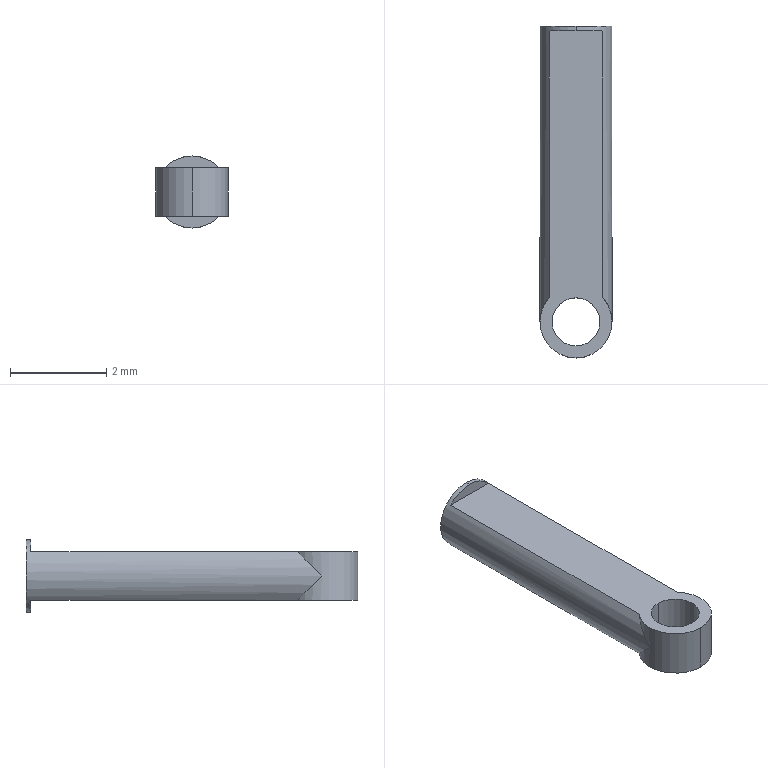Component | SolidWorks | ConnectingRodRockerArm-10 | 1 solid | 17 faces | box 1.5 x 6.9 x 1.5 mm | volume 6 mm3 | cylinder 10 | plane 7 | commonest cylinder face diameters 1.5 x4 1 x2 0.7 x2 0.8 x2
STEP:
#1=COLOUR_RGB('',0.7922,0.8196,0.9333);
#2=FILL_AREA_STYLE_COLOUR('',#1);
#3=FILL_AREA_STYLE('',(#2));
#4=SURFACE_STYLE_FILL_AREA(#3);
#5=SURFACE_SIDE_STYLE('',(#4));
#6=SURFACE_STYLE_USAGE(.BOTH.,#5);
#7=PRESENTATION_STYLE_ASSIGNMENT((#6));
#8=CARTESIAN_POINT('',(0.3877,0.1328,0.2657));
#9=VERTEX_POINT('',#8);
#10=CARTESIAN_POINT('',(0.3877,0.1328,0.3248));
#11=VERTEX_POINT('',#10);
#12=CARTESIAN_POINT('',(0.3877,0.1328,0.2953));
#13=DIRECTION('',(-0.,1.,-0.));
#14=DIRECTION('',(0.,0.,-1.));
#15=AXIS2_PLACEMENT_3D('',#12,#13,#14);
#16=CIRCLE('',#15,0.02953);
#17=EDGE_CURVE('',#9,#11,#16,.T.);
#18=ORIENTED_EDGE('',*,*,#17,.F.);
#19=CARTESIAN_POINT('',(0.3877,0.1289,0.2657));
#20=VERTEX_POINT('',#19);
#21=CARTESIAN_POINT('',(0.3877,0.1289,0.2657));
#22=DIRECTION('',(0.,-1.,0.));
#23=VECTOR('',#22,39.37);
#24=LINE('',#21,#23);
#25=EDGE_CURVE('',#9,#20,#24,.T.);
#26=ORIENTED_EDGE('',*,*,#25,.T.);
#27=CARTESIAN_POINT('',(0.3657,0.1289,0.2756));
#28=VERTEX_POINT('',#27);
#29=CARTESIAN_POINT('',(0.3877,0.1289,0.2953));
#30=DIRECTION('',(-0.,1.,-0.));
#31=DIRECTION('',(0.,0.,-1.));
#32=AXIS2_PLACEMENT_3D('',#29,#30,#31);
#33=CIRCLE('',#32,0.02953);
#34=EDGE_CURVE('',#20,#28,#33,.T.);
#35=ORIENTED_EDGE('',*,*,#34,.T.);
#36=CARTESIAN_POINT('',(0.3657,-0.08962,0.2756));
#37=VERTEX_POINT('',#36);
#38=CARTESIAN_POINT('',(0.3657,0.1289,0.2756));
#39=DIRECTION('',(-0.,1.,-0.));
#40=VECTOR('',#39,39.37);
#41=LINE('',#38,#40);
#42=EDGE_CURVE('',#37,#28,#41,.T.);
#43=ORIENTED_EDGE('',*,*,#42,.F.);
#44=CARTESIAN_POINT('',(0.3581,-0.1093,0.2953));
#45=VERTEX_POINT('',#44);
#46=CARTESIAN_POINT('',(0.3657,-0.08962,0.2756));
#47=CARTESIAN_POINT('',(0.3608,-0.09509,0.2811));
#48=CARTESIAN_POINT('',(0.3581,-0.102,0.2879));
#49=CARTESIAN_POINT('',(0.3581,-0.1093,0.2953));
#50=(BOUNDED_CURVE()B_SPLINE_CURVE(3,(#46,#47,#48,#49),.UNSPECIFIED.,.F.,.F.)B_SPLINE_CURVE_WITH_KNOTS((4,4),(0.8411,1.571),.UNSPECIFIED.)CURVE()GEOMETRIC_REPRESENTATION_ITEM()RATIONAL_B_SPLINE_CURVE((1.,0.9561,0.9561,1.))REPRESENTATION_ITEM(''));
#51=EDGE_CURVE('',#37,#45,#50,.T.);
#52=ORIENTED_EDGE('',*,*,#51,.T.);
#53=CARTESIAN_POINT('',(0.3657,-0.08962,0.315));
#54=VERTEX_POINT('',#53);
#55=CARTESIAN_POINT('',(0.3581,-0.1093,0.2953));
#56=CARTESIAN_POINT('',(0.3581,-0.102,0.3026));
#57=CARTESIAN_POINT('',(0.3608,-0.09509,0.3095));
#58=CARTESIAN_POINT('',(0.3657,-0.08962,0.315));
#59=(BOUNDED_CURVE()B_SPLINE_CURVE(3,(#55,#56,#57,#58),.UNSPECIFIED.,.F.,.T.)B_SPLINE_CURVE_WITH_KNOTS((4,4),(1.571,2.301),.UNSPECIFIED.)CURVE()GEOMETRIC_REPRESENTATION_ITEM()RATIONAL_B_SPLINE_CURVE((1.,0.9561,0.9561,1.))REPRESENTATION_ITEM(''));
#60=EDGE_CURVE('',#45,#54,#59,.T.);
#61=ORIENTED_EDGE('',*,*,#60,.T.);
#62=CARTESIAN_POINT('',(0.3657,0.1289,0.315));
#63=VERTEX_POINT('',#62);
#64=CARTESIAN_POINT('',(0.3657,0.1289,0.315));
#65=DIRECTION('',(0.,-1.,0.));
#66=VECTOR('',#65,39.37);
#67=LINE('',#64,#66);
#68=EDGE_CURVE('',#63,#54,#67,.T.);
#69=ORIENTED_EDGE('',*,*,#68,.F.);
#70=CARTESIAN_POINT('',(0.3877,0.1289,0.3248));
#71=VERTEX_POINT('',#70);
#72=CARTESIAN_POINT('',(0.3877,0.1289,0.2953));
#73=DIRECTION('',(-0.,1.,-0.));
#74=DIRECTION('',(0.,0.,-1.));
#75=AXIS2_PLACEMENT_3D('',#72,#73,#74);
#76=CIRCLE('',#75,0.02953);
#77=EDGE_CURVE('',#63,#71,#76,.T.);
#78=ORIENTED_EDGE('',*,*,#77,.T.);
#79=CARTESIAN_POINT('',(0.3877,0.1289,0.3248));
#80=DIRECTION('',(0.,-1.,0.));
#81=VECTOR('',#80,39.37);
#82=LINE('',#79,#81);
#83=EDGE_CURVE('',#11,#71,#82,.T.);
#84=ORIENTED_EDGE('',*,*,#83,.F.);
#85=EDGE_LOOP('',(#18,#26,#35,#43,#52,#61,#69,#78,#84));
#86=FACE_OUTER_BOUND('',#85,.T.);
#87=CARTESIAN_POINT('',(0.3877,0.1289,0.2953));
#88=DIRECTION('',(0.,-1.,0.));
#89=DIRECTION('',(0.,0.,1.));
#90=AXIS2_PLACEMENT_3D('',#87,#88,#89);
#91=CYLINDRICAL_SURFACE('',#90,0.02953);
#92=ADVANCED_FACE('',(#86),#91,.T.);
#93=CARTESIAN_POINT('',(0.3877,-0.129,0.2756));
#94=VERTEX_POINT('',#93);
#95=CARTESIAN_POINT('',(0.3877,-0.08962,0.2756));
#96=VERTEX_POINT('',#95);
#97=CARTESIAN_POINT('',(0.3877,-0.1093,0.2756));
#98=DIRECTION('',(-0.,-0.,1.));
#99=DIRECTION('',(0.,1.,0.));
#100=AXIS2_PLACEMENT_3D('',#97,#98,#99);
#101=CIRCLE('',#100,0.01969);
#102=EDGE_CURVE('',#94,#96,#101,.T.);
#103=ORIENTED_EDGE('',*,*,#102,.F.);
#104=CARTESIAN_POINT('',(0.3877,-0.129,0.315));
#105=VERTEX_POINT('',#104);
#106=CARTESIAN_POINT('',(0.3877,-0.129,0.2756));
#107=DIRECTION('',(-0.,-0.,1.));
#108=VECTOR('',#107,39.37);
#109=LINE('',#106,#108);
#110=EDGE_CURVE('',#94,#105,#109,.T.);
#111=ORIENTED_EDGE('',*,*,#110,.T.);
#112=CARTESIAN_POINT('',(0.3877,-0.08962,0.315));
#113=VERTEX_POINT('',#112);
#114=CARTESIAN_POINT('',(0.3877,-0.1093,0.315));
#115=DIRECTION('',(-0.,-0.,1.));
#116=DIRECTION('',(0.,1.,0.));
#117=AXIS2_PLACEMENT_3D('',#114,#115,#116);
#118=CIRCLE('',#117,0.01969);
#119=EDGE_CURVE('',#105,#113,#118,.T.);
#120=ORIENTED_EDGE('',*,*,#119,.T.);
#121=CARTESIAN_POINT('',(0.3877,-0.08962,0.2756));
#122=DIRECTION('',(-0.,-0.,1.));
#123=VECTOR('',#122,39.37);
#124=LINE('',#121,#123);
#125=EDGE_CURVE('',#96,#113,#124,.T.);
#126=ORIENTED_EDGE('',*,*,#125,.F.);
#127=EDGE_LOOP('',(#103,#111,#120,#126));
#128=FACE_OUTER_BOUND('',#127,.T.);
#129=CARTESIAN_POINT('',(0.3877,-0.1093,0.2756));
#130=DIRECTION('',(-0.,-0.,1.));
#131=DIRECTION('',(0.,1.,0.));
#132=AXIS2_PLACEMENT_3D('',#129,#130,#131);
#133=CYLINDRICAL_SURFACE('',#132,0.01969);
#134=ADVANCED_FACE('',(#128),#133,.F.);
#135=CARTESIAN_POINT('',(0.3877,-0.1388,0.315));
#136=VERTEX_POINT('',#135);
#137=CARTESIAN_POINT('',(0.4097,-0.08962,0.315));
#138=VERTEX_POINT('',#137);
#139=CARTESIAN_POINT('',(0.3877,-0.1093,0.315));
#140=DIRECTION('',(-0.,-0.,1.));
#141=DIRECTION('',(0.,1.,0.));
#142=AXIS2_PLACEMENT_3D('',#139,#140,#141);
#143=CIRCLE('',#142,0.02953);
#144=EDGE_CURVE('',#136,#138,#143,.T.);
#145=ORIENTED_EDGE('',*,*,#144,.F.);
#146=CARTESIAN_POINT('',(0.3877,-0.1388,0.2756));
#147=VERTEX_POINT('',#146);
#148=CARTESIAN_POINT('',(0.3877,-0.1388,0.315));
#149=DIRECTION('',(0.,0.,-1.));
#150=VECTOR('',#149,39.37);
#151=LINE('',#148,#150);
#152=EDGE_CURVE('',#136,#147,#151,.T.);
#153=ORIENTED_EDGE('',*,*,#152,.T.);
#154=CARTESIAN_POINT('',(0.4097,-0.08962,0.2756));
#155=VERTEX_POINT('',#154);
#156=CARTESIAN_POINT('',(0.3877,-0.1093,0.2756));
#157=DIRECTION('',(-0.,-0.,1.));
#158=DIRECTION('',(0.,1.,0.));
#159=AXIS2_PLACEMENT_3D('',#156,#157,#158);
#160=CIRCLE('',#159,0.02953);
#161=EDGE_CURVE('',#147,#155,#160,.T.);
#162=ORIENTED_EDGE('',*,*,#161,.T.);
#163=CARTESIAN_POINT('',(0.4172,-0.1093,0.2953));
#164=VERTEX_POINT('',#163);
#165=CARTESIAN_POINT('',(0.4172,-0.1093,0.2953));
#166=CARTESIAN_POINT('',(0.4172,-0.102,0.2879));
#167=CARTESIAN_POINT('',(0.4146,-0.09509,0.2811));
#168=CARTESIAN_POINT('',(0.4097,-0.08962,0.2756));
#169=(BOUNDED_CURVE()B_SPLINE_CURVE(3,(#165,#166,#167,#168),.UNSPECIFIED.,.F.,.T.)B_SPLINE_CURVE_WITH_KNOTS((4,4),(4.712,5.442),.UNSPECIFIED.)CURVE()GEOMETRIC_REPRESENTATION_ITEM()RATIONAL_B_SPLINE_CURVE((1.,0.9561,0.9561,1.))REPRESENTATION_ITEM(''));
#170=EDGE_CURVE('',#164,#155,#169,.T.);
#171=ORIENTED_EDGE('',*,*,#170,.F.);
#172=CARTESIAN_POINT('',(0.4097,-0.08962,0.315));
#173=CARTESIAN_POINT('',(0.4146,-0.09509,0.3095));
#174=CARTESIAN_POINT('',(0.4172,-0.102,0.3026));
#175=CARTESIAN_POINT('',(0.4172,-0.1093,0.2953));
#176=(BOUNDED_CURVE()B_SPLINE_CURVE(3,(#172,#173,#174,#175),.UNSPECIFIED.,.F.,.F.)B_SPLINE_CURVE_WITH_KNOTS((4,4),(3.983,4.712),.UNSPECIFIED.)CURVE()GEOMETRIC_REPRESENTATION_ITEM()RATIONAL_B_SPLINE_CURVE((1.,0.9561,0.9561,1.))REPRESENTATION_ITEM(''));
#177=EDGE_CURVE('',#138,#164,#176,.T.);
#178=ORIENTED_EDGE('',*,*,#177,.F.);
#179=EDGE_LOOP('',(#145,#153,#162,#171,#178));
#180=FACE_OUTER_BOUND('',#179,.T.);
#181=CARTESIAN_POINT('',(0.3877,-0.1093,0.315));
#182=DIRECTION('',(0.,0.,-1.));
#183=DIRECTION('',(0.,-1.,0.));
#184=AXIS2_PLACEMENT_3D('',#181,#182,#183);
#185=CYLINDRICAL_SURFACE('',#184,0.02953);
#186=ADVANCED_FACE('',(#180),#185,.T.);
#187=CARTESIAN_POINT('',(0.3877,0.1328,0.3091));
#188=VERTEX_POINT('',#187);
#189=CARTESIAN_POINT('',(0.3877,0.1328,0.2815));
#190=VERTEX_POINT('',#189);
#191=CARTESIAN_POINT('',(0.3877,0.1328,0.2953));
#192=DIRECTION('',(-0.,1.,-0.));
#193=DIRECTION('',(0.,0.,-1.));
#194=AXIS2_PLACEMENT_3D('',#191,#192,#193);
#195=CIRCLE('',#194,0.01378);
#196=EDGE_CURVE('',#188,#190,#195,.T.);
#197=ORIENTED_EDGE('',*,*,#196,.T.);
#198=CARTESIAN_POINT('',(0.3877,0.1289,0.2815));
#199=VERTEX_POINT('',#198);
#200=CARTESIAN_POINT('',(0.3877,0.1328,0.2815));
#201=DIRECTION('',(0.,-1.,0.));
#202=VECTOR('',#201,39.37);
#203=LINE('',#200,#202);
#204=EDGE_CURVE('',#190,#199,#203,.T.);
#205=ORIENTED_EDGE('',*,*,#204,.T.);
#206=CARTESIAN_POINT('',(0.3877,0.1289,0.3091));
#207=VERTEX_POINT('',#206);
#208=CARTESIAN_POINT('',(0.3877,0.1289,0.2953));
#209=DIRECTION('',(-0.,1.,-0.));
#210=DIRECTION('',(0.,0.,-1.));
#211=AXIS2_PLACEMENT_3D('',#208,#209,#210);
#212=CIRCLE('',#211,0.01378);
#213=EDGE_CURVE('',#207,#199,#212,.T.);
#214=ORIENTED_EDGE('',*,*,#213,.F.);
#215=CARTESIAN_POINT('',(0.3877,0.1328,0.3091));
#216=DIRECTION('',(0.,-1.,0.));
#217=VECTOR('',#216,39.37);
#218=LINE('',#215,#217);
#219=EDGE_CURVE('',#188,#207,#218,.T.);
#220=ORIENTED_EDGE('',*,*,#219,.F.);
#221=EDGE_LOOP('',(#197,#205,#214,#220));
#222=FACE_OUTER_BOUND('',#221,.T.);
#223=CARTESIAN_POINT('',(0.3877,0.1328,0.2953));
#224=DIRECTION('',(0.,-1.,0.));
#225=DIRECTION('',(0.,0.,1.));
#226=AXIS2_PLACEMENT_3D('',#223,#224,#225);
#227=CYLINDRICAL_SURFACE('',#226,0.01378);
#228=ADVANCED_FACE('',(#222),#227,.F.);
#229=CARTESIAN_POINT('',(0.3877,-0.06797,0.311));
#230=VERTEX_POINT('',#229);
#231=CARTESIAN_POINT('',(0.3877,-0.06797,0.2795));
#232=VERTEX_POINT('',#231);
#233=CARTESIAN_POINT('',(0.3877,-0.06797,0.2953));
#234=DIRECTION('',(-0.,1.,-0.));
#235=DIRECTION('',(0.,0.,-1.));
#236=AXIS2_PLACEMENT_3D('',#233,#234,#235);
#237=CIRCLE('',#236,0.01575);
#238=EDGE_CURVE('',#230,#232,#237,.T.);
#239=ORIENTED_EDGE('',*,*,#238,.F.);
#240=CARTESIAN_POINT('',(0.3877,0.1289,0.311));
#241=VERTEX_POINT('',#240);
#242=CARTESIAN_POINT('',(0.3877,-0.06797,0.311));
#243=DIRECTION('',(-0.,1.,-0.));
#244=VECTOR('',#243,39.37);
#245=LINE('',#242,#244);
#246=EDGE_CURVE('',#230,#241,#245,.T.);
#247=ORIENTED_EDGE('',*,*,#246,.T.);
#248=CARTESIAN_POINT('',(0.3877,0.1289,0.2795));
#249=VERTEX_POINT('',#248);
#250=CARTESIAN_POINT('',(0.3877,0.1289,0.2953));
#251=DIRECTION('',(-0.,1.,-0.));
#252=DIRECTION('',(0.,0.,-1.));
#253=AXIS2_PLACEMENT_3D('',#250,#251,#252);
#254=CIRCLE('',#253,0.01575);
#255=EDGE_CURVE('',#241,#249,#254,.T.);
#256=ORIENTED_EDGE('',*,*,#255,.T.);
#257=CARTESIAN_POINT('',(0.3877,-0.06797,0.2795));
#258=DIRECTION('',(-0.,1.,-0.));
#259=VECTOR('',#258,39.37);
#260=LINE('',#257,#259);
#261=EDGE_CURVE('',#232,#249,#260,.T.);
#262=ORIENTED_EDGE('',*,*,#261,.F.);
#263=EDGE_LOOP('',(#239,#247,#256,#262));
#264=FACE_OUTER_BOUND('',#263,.T.);
#265=CARTESIAN_POINT('',(0.3877,-0.06797,0.2953));
#266=DIRECTION('',(-0.,1.,-0.));
#267=DIRECTION('',(0.,0.,-1.));
#268=AXIS2_PLACEMENT_3D('',#265,#266,#267);
#269=CYLINDRICAL_SURFACE('',#268,0.01575);
#270=ADVANCED_FACE('',(#264),#269,.F.);
#271=ORIENTED_EDGE('',*,*,#246,.F.);
#272=CARTESIAN_POINT('',(0.3877,-0.06797,0.2953));
#273=DIRECTION('',(-0.,1.,-0.));
#274=DIRECTION('',(0.,0.,-1.));
#275=AXIS2_PLACEMENT_3D('',#272,#273,#274);
#276=CIRCLE('',#275,0.01575);
#277=EDGE_CURVE('',#232,#230,#276,.T.);
#278=ORIENTED_EDGE('',*,*,#277,.F.);
#279=ORIENTED_EDGE('',*,*,#261,.T.);
#280=CARTESIAN_POINT('',(0.3877,0.1289,0.2953));
#281=DIRECTION('',(-0.,1.,-0.));
#282=DIRECTION('',(0.,0.,-1.));
#283=AXIS2_PLACEMENT_3D('',#280,#281,#282);
#284=CIRCLE('',#283,0.01575);
#285=EDGE_CURVE('',#249,#241,#284,.T.);
#286=ORIENTED_EDGE('',*,*,#285,.T.);
#287=EDGE_LOOP('',(#271,#278,#279,#286));
#288=FACE_OUTER_BOUND('',#287,.T.);
#289=CARTESIAN_POINT('',(0.3877,-0.06797,0.2953));
#290=DIRECTION('',(-0.,1.,-0.));
#291=DIRECTION('',(0.,0.,-1.));
#292=AXIS2_PLACEMENT_3D('',#289,#290,#291);
#293=CYLINDRICAL_SURFACE('',#292,0.01575);
#294=ADVANCED_FACE('',(#288),#293,.F.);
#295=ORIENTED_EDGE('',*,*,#277,.T.);
#296=ORIENTED_EDGE('',*,*,#238,.T.);
#297=EDGE_LOOP('',(#295,#296));
#298=FACE_OUTER_BOUND('',#297,.T.);
#299=CARTESIAN_POINT('',(0.3877,-0.06797,0.2953));
#300=DIRECTION('',(-0.,1.,0.));
#301=DIRECTION('',(0.,0.,-1.));
#302=AXIS2_PLACEMENT_3D('',#299,#300,#301);
#303=PLANE('',#302);
#304=ADVANCED_FACE('',(#298),#303,.T.);
#305=CARTESIAN_POINT('',(0.4097,0.1289,0.2756));
#306=VERTEX_POINT('',#305);
#307=CARTESIAN_POINT('',(0.3877,0.1289,0.2953));
#308=DIRECTION('',(-0.,1.,-0.));
#309=DIRECTION('',(0.,0.,-1.));
#310=AXIS2_PLACEMENT_3D('',#307,#308,#309);
#311=CIRCLE('',#310,0.02953);
#312=EDGE_CURVE('',#306,#20,#311,.T.);
#313=ORIENTED_EDGE('',*,*,#312,.F.);
#314=CARTESIAN_POINT('',(0.4172,0.1289,0.2756));
#315=DIRECTION('',(-1.,-0.,-0.));
#316=VECTOR('',#315,39.37);
#317=LINE('',#314,#316);
#318=EDGE_CURVE('',#306,#28,#317,.T.);
#319=ORIENTED_EDGE('',*,*,#318,.T.);
#320=ORIENTED_EDGE('',*,*,#34,.F.);
#321=EDGE_LOOP('',(#313,#319,#320));
#322=FACE_OUTER_BOUND('',#321,.T.);
#323=CARTESIAN_POINT('',(0.3877,0.1289,0.2953));
#324=DIRECTION('',(-0.,1.,0.));
#325=DIRECTION('',(0.,0.,-1.));
#326=AXIS2_PLACEMENT_3D('',#323,#324,#325);
#327=PLANE('',#326);
#328=ADVANCED_FACE('',(#322),#327,.F.);
#329=ORIENTED_EDGE('',*,*,#77,.F.);
#330=CARTESIAN_POINT('',(0.4097,0.1289,0.315));
#331=VERTEX_POINT('',#330);
#332=CARTESIAN_POINT('',(0.4172,0.1289,0.315));
#333=DIRECTION('',(1.,0.,0.));
#334=VECTOR('',#333,39.37);
#335=LINE('',#332,#334);
#336=EDGE_CURVE('',#63,#331,#335,.T.);
#337=ORIENTED_EDGE('',*,*,#336,.T.);
#338=CARTESIAN_POINT('',(0.3877,0.1289,0.2953));
#339=DIRECTION('',(-0.,1.,-0.));
#340=DIRECTION('',(0.,0.,-1.));
#341=AXIS2_PLACEMENT_3D('',#338,#339,#340);
#342=CIRCLE('',#341,0.02953);
#343=EDGE_CURVE('',#71,#331,#342,.T.);
#344=ORIENTED_EDGE('',*,*,#343,.F.);
#345=EDGE_LOOP('',(#329,#337,#344));
#346=FACE_OUTER_BOUND('',#345,.T.);
#347=CARTESIAN_POINT('',(0.3877,0.1289,0.2953));
#348=DIRECTION('',(-0.,1.,0.));
#349=DIRECTION('',(0.,0.,-1.));
#350=AXIS2_PLACEMENT_3D('',#347,#348,#349);
#351=PLANE('',#350);
#352=ADVANCED_FACE('',(#346),#351,.F.);
#353=CARTESIAN_POINT('',(0.3877,0.1328,0.2953));
#354=DIRECTION('',(-0.,1.,-0.));
#355=DIRECTION('',(0.,0.,-1.));
#356=AXIS2_PLACEMENT_3D('',#353,#354,#355);
#357=CIRCLE('',#356,0.02953);
#358=EDGE_CURVE('',#11,#9,#357,.T.);
#359=ORIENTED_EDGE('',*,*,#358,.T.);
#360=ORIENTED_EDGE('',*,*,#17,.T.);
#361=EDGE_LOOP('',(#359,#360));
#362=FACE_OUTER_BOUND('',#361,.T.);
#363=ORIENTED_EDGE('',*,*,#196,.F.);
#364=CARTESIAN_POINT('',(0.3877,0.1328,0.2953));
#365=DIRECTION('',(-0.,1.,-0.));
#366=DIRECTION('',(0.,0.,-1.));
#367=AXIS2_PLACEMENT_3D('',#364,#365,#366);
#368=CIRCLE('',#367,0.01378);
#369=EDGE_CURVE('',#190,#188,#368,.T.);
#370=ORIENTED_EDGE('',*,*,#369,.F.);
#371=EDGE_LOOP('',(#363,#370));
#372=FACE_BOUND('',#371,.T.);
#373=CARTESIAN_POINT('',(0.3877,0.1328,0.2953));
#374=DIRECTION('',(-0.,1.,0.));
#375=DIRECTION('',(0.,0.,-1.));
#376=AXIS2_PLACEMENT_3D('',#373,#374,#375);
#377=PLANE('',#376);
#378=ADVANCED_FACE('',(#362,#372),#377,.T.);
#379=ORIENTED_EDGE('',*,*,#285,.F.);
#380=ORIENTED_EDGE('',*,*,#255,.F.);
#381=EDGE_LOOP('',(#379,#380));
#382=FACE_OUTER_BOUND('',#381,.T.);
#383=ORIENTED_EDGE('',*,*,#213,.T.);
#384=CARTESIAN_POINT('',(0.3877,0.1289,0.2953));
#385=DIRECTION('',(-0.,1.,-0.));
#386=DIRECTION('',(0.,0.,-1.));
#387=AXIS2_PLACEMENT_3D('',#384,#385,#386);
#388=CIRCLE('',#387,0.01378);
#389=EDGE_CURVE('',#199,#207,#388,.T.);
#390=ORIENTED_EDGE('',*,*,#389,.T.);
#391=EDGE_LOOP('',(#383,#390));
#392=FACE_BOUND('',#391,.T.);
#393=CARTESIAN_POINT('',(0.3877,0.1289,0.2953));
#394=DIRECTION('',(-0.,1.,0.));
#395=DIRECTION('',(0.,0.,-1.));
#396=AXIS2_PLACEMENT_3D('',#393,#394,#395);
#397=PLANE('',#396);
#398=ADVANCED_FACE('',(#382,#392),#397,.F.);
#399=ORIENTED_EDGE('',*,*,#204,.F.);
#400=ORIENTED_EDGE('',*,*,#369,.T.);
#401=ORIENTED_EDGE('',*,*,#219,.T.);
#402=ORIENTED_EDGE('',*,*,#389,.F.);
#403=EDGE_LOOP('',(#399,#400,#401,#402));
#404=FACE_OUTER_BOUND('',#403,.T.);
#405=CARTESIAN_POINT('',(0.3877,0.1328,0.2953));
#406=DIRECTION('',(0.,-1.,0.));
#407=DIRECTION('',(0.,0.,1.));
#408=AXIS2_PLACEMENT_3D('',#405,#406,#407);
#409=CYLINDRICAL_SURFACE('',#408,0.01378);
#410=ADVANCED_FACE('',(#404),#409,.F.);
#411=ORIENTED_EDGE('',*,*,#152,.F.);
#412=CARTESIAN_POINT('',(0.3877,-0.1093,0.315));
#413=DIRECTION('',(-0.,-0.,1.));
#414=DIRECTION('',(0.,1.,0.));
#415=AXIS2_PLACEMENT_3D('',#412,#413,#414);
#416=CIRCLE('',#415,0.02953);
#417=EDGE_CURVE('',#54,#136,#416,.T.);
#418=ORIENTED_EDGE('',*,*,#417,.F.);
#419=ORIENTED_EDGE('',*,*,#60,.F.);
#420=ORIENTED_EDGE('',*,*,#51,.F.);
#421=CARTESIAN_POINT('',(0.3877,-0.1093,0.2756));
#422=DIRECTION('',(-0.,-0.,1.));
#423=DIRECTION('',(0.,1.,0.));
#424=AXIS2_PLACEMENT_3D('',#421,#422,#423);
#425=CIRCLE('',#424,0.02953);
#426=EDGE_CURVE('',#37,#147,#425,.T.);
#427=ORIENTED_EDGE('',*,*,#426,.T.);
#428=EDGE_LOOP('',(#411,#418,#419,#420,#427));
#429=FACE_OUTER_BOUND('',#428,.T.);
#430=CARTESIAN_POINT('',(0.3877,-0.1093,0.315));
#431=DIRECTION('',(0.,0.,-1.));
#432=DIRECTION('',(0.,-1.,0.));
#433=AXIS2_PLACEMENT_3D('',#430,#431,#432);
#434=CYLINDRICAL_SURFACE('',#433,0.02953);
#435=ADVANCED_FACE('',(#429),#434,.T.);
#436=ORIENTED_EDGE('',*,*,#110,.F.);
#437=CARTESIAN_POINT('',(0.3877,-0.1093,0.2756));
#438=DIRECTION('',(-0.,-0.,1.));
#439=DIRECTION('',(0.,1.,0.));
#440=AXIS2_PLACEMENT_3D('',#437,#438,#439);
#441=CIRCLE('',#440,0.01969);
#442=EDGE_CURVE('',#96,#94,#441,.T.);
#443=ORIENTED_EDGE('',*,*,#442,.F.);
#444=ORIENTED_EDGE('',*,*,#125,.T.);
#445=CARTESIAN_POINT('',(0.3877,-0.1093,0.315));
#446=DIRECTION('',(-0.,-0.,1.));
#447=DIRECTION('',(0.,1.,0.));
#448=AXIS2_PLACEMENT_3D('',#445,#446,#447);
#449=CIRCLE('',#448,0.01969);
#450=EDGE_CURVE('',#113,#105,#449,.T.);
#451=ORIENTED_EDGE('',*,*,#450,.T.);
#452=EDGE_LOOP('',(#436,#443,#444,#451));
#453=FACE_OUTER_BOUND('',#452,.T.);
#454=CARTESIAN_POINT('',(0.3877,-0.1093,0.2756));
#455=DIRECTION('',(-0.,-0.,1.));
#456=DIRECTION('',(0.,1.,0.));
#457=AXIS2_PLACEMENT_3D('',#454,#455,#456);
#458=CYLINDRICAL_SURFACE('',#457,0.01969);
#459=ADVANCED_FACE('',(#453),#458,.F.);
#460=ORIENTED_EDGE('',*,*,#442,.T.);
#461=ORIENTED_EDGE('',*,*,#102,.T.);
#462=EDGE_LOOP('',(#460,#461));
#463=FACE_BOUND('',#462,.T.);
#464=CARTESIAN_POINT('',(0.4097,0.1289,0.2756));
#465=DIRECTION('',(0.,-1.,0.));
#466=VECTOR('',#465,39.37);
#467=LINE('',#464,#466);
#468=EDGE_CURVE('',#306,#155,#467,.T.);
#469=ORIENTED_EDGE('',*,*,#468,.T.);
#470=ORIENTED_EDGE('',*,*,#161,.F.);
#471=ORIENTED_EDGE('',*,*,#426,.F.);
#472=ORIENTED_EDGE('',*,*,#42,.T.);
#473=ORIENTED_EDGE('',*,*,#318,.F.);
#474=EDGE_LOOP('',(#469,#470,#471,#472,#473));
#475=FACE_OUTER_BOUND('',#474,.T.);
#476=CARTESIAN_POINT('',(0.3877,-0.1093,0.2756));
#477=DIRECTION('',(-0.,0.,1.));
#478=DIRECTION('',(-0.,1.,-0.));
#479=AXIS2_PLACEMENT_3D('',#476,#477,#478);
#480=PLANE('',#479);
#481=ADVANCED_FACE('',(#463,#475),#480,.F.);
#482=ORIENTED_EDGE('',*,*,#450,.F.);
#483=ORIENTED_EDGE('',*,*,#119,.F.);
#484=EDGE_LOOP('',(#482,#483));
#485=FACE_BOUND('',#484,.T.);
#486=ORIENTED_EDGE('',*,*,#417,.T.);
#487=ORIENTED_EDGE('',*,*,#144,.T.);
#488=CARTESIAN_POINT('',(0.4097,0.1289,0.315));
#489=DIRECTION('',(-0.,1.,-0.));
#490=VECTOR('',#489,39.37);
#491=LINE('',#488,#490);
#492=EDGE_CURVE('',#138,#331,#491,.T.);
#493=ORIENTED_EDGE('',*,*,#492,.T.);
#494=ORIENTED_EDGE('',*,*,#336,.F.);
#495=ORIENTED_EDGE('',*,*,#68,.T.);
#496=EDGE_LOOP('',(#486,#487,#493,#494,#495));
#497=FACE_OUTER_BOUND('',#496,.T.);
#498=CARTESIAN_POINT('',(0.3877,-0.1093,0.315));
#499=DIRECTION('',(-0.,0.,1.));
#500=DIRECTION('',(-0.,1.,-0.));
#501=AXIS2_PLACEMENT_3D('',#498,#499,#500);
#502=PLANE('',#501);
#503=ADVANCED_FACE('',(#485,#497),#502,.T.);
#504=ORIENTED_EDGE('',*,*,#25,.F.);
#505=ORIENTED_EDGE('',*,*,#358,.F.);
#506=ORIENTED_EDGE('',*,*,#83,.T.);
#507=ORIENTED_EDGE('',*,*,#343,.T.);
#508=ORIENTED_EDGE('',*,*,#492,.F.);
#509=ORIENTED_EDGE('',*,*,#177,.T.);
#510=ORIENTED_EDGE('',*,*,#170,.T.);
#511=ORIENTED_EDGE('',*,*,#468,.F.);
#512=ORIENTED_EDGE('',*,*,#312,.T.);
#513=EDGE_LOOP('',(#504,#505,#506,#507,#508,#509,#510,#511,#512));
#514=FACE_OUTER_BOUND('',#513,.T.);
#515=CARTESIAN_POINT('',(0.3877,0.1289,0.2953));
#516=DIRECTION('',(0.,-1.,0.));
#517=DIRECTION('',(0.,0.,1.));
#518=AXIS2_PLACEMENT_3D('',#515,#516,#517);
#519=CYLINDRICAL_SURFACE('',#518,0.02953);
#520=ADVANCED_FACE('',(#514),#519,.T.);
#521=CLOSED_SHELL('',(#92,#134,#186,#228,#270,#294,#304,#328,#352,#378,#398,#410,#435,#459,#481,#503,#520));
#522=MANIFOLD_SOLID_BREP('',#521);
#523=STYLED_ITEM('',(#7),#522);
#524=(LENGTH_UNIT()NAMED_UNIT(*)SI_UNIT($,.METRE.));
#525=LENGTH_MEASURE_WITH_UNIT(LENGTH_MEASURE(0.0254),#524);
#526=DIMENSIONAL_EXPONENTS(1.,0.,0.,0.,0.,0.,0.);
#527=(CONVERSION_BASED_UNIT('',#525)LENGTH_UNIT()NAMED_UNIT(#526));
#528=UNCERTAINTY_MEASURE_WITH_UNIT(LENGTH_MEASURE(0.00001),#527,'','');
#529=(NAMED_UNIT(*)PLANE_ANGLE_UNIT()SI_UNIT($,.RADIAN.));
#530=(NAMED_UNIT(*)SI_UNIT($,.STERADIAN.)SOLID_ANGLE_UNIT());
#531=(GEOMETRIC_REPRESENTATION_CONTEXT(3)GLOBAL_UNCERTAINTY_ASSIGNED_CONTEXT((#528))GLOBAL_UNIT_ASSIGNED_CONTEXT((#527,#529,#530))REPRESENTATION_CONTEXT('',''));
#532=MECHANICAL_DESIGN_GEOMETRIC_PRESENTATION_REPRESENTATION('',(#523),#531);
#533=CARTESIAN_POINT('',(0.,0.,0.));
#534=DIRECTION('',(0.,0.,1.));
#535=DIRECTION('',(1.,0.,0.));
#536=AXIS2_PLACEMENT_3D('',#533,#534,#535);
#537=(LENGTH_UNIT()NAMED_UNIT(*)SI_UNIT($,.METRE.));
#538=LENGTH_MEASURE_WITH_UNIT(LENGTH_MEASURE(0.0254),#537);
#539=DIMENSIONAL_EXPONENTS(1.,0.,0.,0.,0.,0.,0.);
#540=(CONVERSION_BASED_UNIT('',#538)LENGTH_UNIT()NAMED_UNIT(#539));
#541=UNCERTAINTY_MEASURE_WITH_UNIT(LENGTH_MEASURE(0.00001),#540,'','');
#542=(NAMED_UNIT(*)PLANE_ANGLE_UNIT()SI_UNIT($,.RADIAN.));
#543=(NAMED_UNIT(*)SI_UNIT($,.STERADIAN.)SOLID_ANGLE_UNIT());
#544=(GEOMETRIC_REPRESENTATION_CONTEXT(3)GLOBAL_UNCERTAINTY_ASSIGNED_CONTEXT((#541))GLOBAL_UNIT_ASSIGNED_CONTEXT((#540,#542,#543))REPRESENTATION_CONTEXT('',''));
#545=ADVANCED_BREP_SHAPE_REPRESENTATION('',(#522,#536),#544);
#546=PRESENTATION_LAYER_ASSIGNMENT('','',(#523));